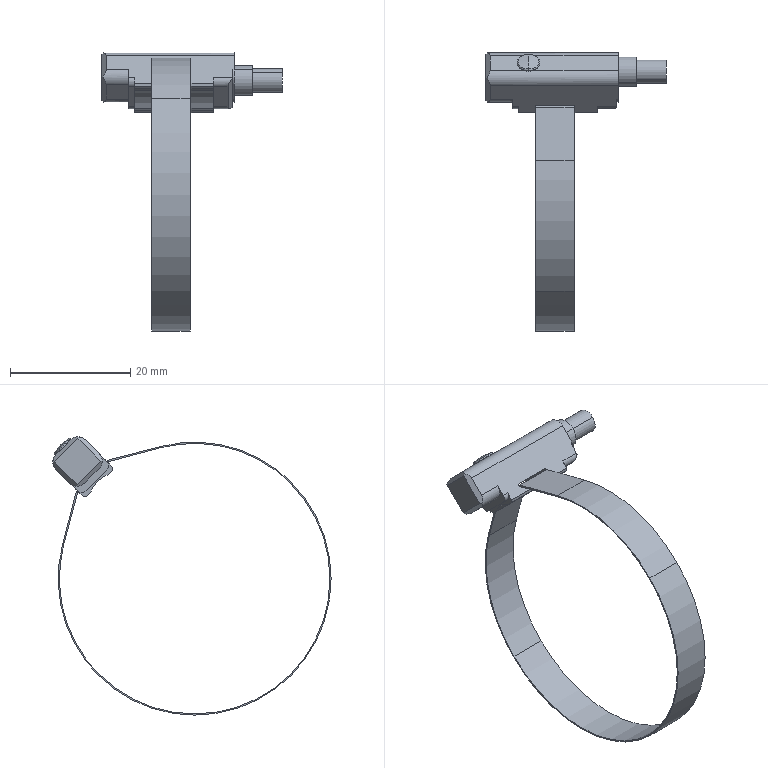Component | SolidWorks | CS1_M_A40-1 | 1 solid | 66 faces | box 30 x 46.28 x 46.28 mm | volume 1437 mm3 | plane 37 | cylinder 25 | sphere 2 | torus 2 | commonest cylinder face diameters 3.4 x6 45 x5 2 x4 45.4 x3 3.8 x2 3.9 x2 4.9 x2 10 x1
build123d program:
from build123d import *

# Parameters (mm, degrees)
EXTRUDE1_DEPTH              = 3.175
EXTRUDE1_DEPTH_BACK         = 3.175
EXTRUDE2_DEPTH              = 18.5
EXTRUDE3_DEPTH              = 4.5
EXTRUDE4_DEPTH              = 5.5
EXTRUDE5_DEPTH              = 18.5
EXTRUDE6_DEPTH              = 3.5
EXTRUDE7_DEPTH              = 3.25
EXTRUDE7_DEPTH_BACK         = 3.25
SKETCH7_W                   = 7.3
SKETCH7_H                   = 0.3
SKETCH8_R                   = 2.45
EXTRUDE8_DEPTH              = 25
SKETCH9_R                   = 1.95
EXTRUDE9_DEPTH              = 30
EXTRUDE10_DEPTH             = 3.2
EXTRUDE11_DEPTH             = 5
EXTRUDE11_DEPTH_BACK        = 5
EXTRUDE12_DEPTH             = 5
EXTRUDE12_DEPTH_BACK        = 5
EXTRUDE13_DEPTH             = 10
EXTRUDE13_DEPTH_BACK        = 10
TUBESADDLERELIEF_DEPTH      = 50.067
TUBESADDLERELIEF_DEPTH_BACK = 50.067
SKETCH15_R                  = 22.5


with BuildPart() as part:
    # Sketch1 → Extrude1 (new, two sides: drawn at the far end of the back side and taken through both)
    with BuildSketch(Plane(origin=(11.5, 0, 0), x_dir=(0, 0, -1), z_dir=(1, 0, 0)).offset(-EXTRUDE1_DEPTH_BACK)):
        with BuildLine():
            Line((11.53, 19.554), (3.65, 24.2))
            Line((3.65, 24.2), (-3.65, 24.2))
            Line((-3.65, 24.2), (-11.53, 19.554))
            ThreePointArc((-11.53, 19.554), (0, -22.7), (11.53, 19.554))
        make_face()
        with BuildLine():
            Line((11.271, 19.474), (3.45, 24))
            Line((3.45, 24), (-3.45, 24))
            Line((-3.45, 24), (-11.271, 19.474))
            ThreePointArc((-11.271, 19.474), (0, -22.5), (11.271, 19.474))
        make_face(mode=Mode.SUBTRACT)
    extrude(amount=EXTRUDE1_DEPTH + EXTRUDE1_DEPTH_BACK)

    # Sketch2 → Extrude2 (add)
    with BuildSketch(Plane(origin=(0, 0, 0), x_dir=(0, 0, -1), z_dir=(1, 0, 0))):
        with BuildLine():
            Line((-3.45, 22.714), (-3.096, 22.361))
            Line((-3.096, 22.361), (-2.5, 22.361))
            Line((-2.5, 22.361), (-2.5, 21.8))
            Line((-2.5, 21.8), (2.5, 21.8))
            Line((2.5, 21.8), (2.5, 22.361))
            Line((2.5, 22.361), (3.096, 22.361))
            Line((3.096, 22.361), (3.45, 22.714))
            Line((3.45, 22.714), (3.45, 29.2))
            ThreePointArc((3.45, 29.2), (2.952, 30.402), (1.75, 30.9))
            Line((1.75, 30.9), (-1.75, 30.9))
            ThreePointArc((-1.75, 30.9), (-2.952, 30.402), (-3.45, 29.2))
            Line((-3.45, 29.2), (-3.45, 22.714))
        make_face()
    extrude(amount=EXTRUDE2_DEPTH)

    # Sketch3 → Extrude3 (cut)
    with BuildSketch(Plane(origin=(0, 0, 0), x_dir=(0, 0, -1), z_dir=(1, 0, 0))):
        with BuildLine():
            Line((-3.45, 25.9), (-3.45, 22.714))
            Line((-3.45, 22.714), (-3.096, 22.361))
            Line((-3.096, 22.361), (-2.5, 22.361))
            Line((-2.5, 22.361), (-2.5, 21.8))
            Line((-2.5, 21.8), (2.5, 21.8))
            Line((2.5, 21.8), (2.5, 22.361))
            Line((2.5, 22.361), (3.096, 22.361))
            Line((3.096, 22.361), (3.45, 22.714))
            Line((3.45, 22.714), (3.45, 25.9))
            ThreePointArc((3.45, 25.9), (2.952, 24.698), (1.75, 24.2))
            Line((1.75, 24.2), (-1.75, 24.2))
            ThreePointArc((-1.75, 24.2), (-2.952, 24.698), (-3.45, 25.9))
        make_face()
    extrude(amount=EXTRUDE3_DEPTH, mode=Mode.SUBTRACT)

    # Sketch4 → Extrude4 (cut)
    with BuildSketch(Plane(origin=(0, 0, 0), x_dir=(0, 0, -1), z_dir=(1, 0, 0))):
        with BuildLine():
            Line((-3.45, 22.714), (-3.096, 22.361))
            Line((-3.096, 22.361), (-2.5, 22.361))
            Line((-2.5, 22.361), (-2.5, 21.8))
            Line((-2.5, 21.8), (2.5, 21.8))
            Line((2.5, 21.8), (2.5, 22.361))
            Line((2.5, 22.361), (3.096, 22.361))
            Line((3.096, 22.361), (3.45, 22.714))
            Line((3.45, 22.714), (3.45, 24.1))
            ThreePointArc((3.45, 24.1), (3.157, 23.393), (2.45, 23.1))
            Line((2.45, 23.1), (-2.45, 23.1))
            ThreePointArc((-2.45, 23.1), (-3.157, 23.393), (-3.45, 24.1))
            Line((-3.45, 24.1), (-3.45, 22.714))
        make_face()
    extrude(amount=EXTRUDE4_DEPTH, mode=Mode.SUBTRACT)

    # Sketch5 → Extrude5 (cut)
    with BuildSketch(Plane(origin=(0, 0, 0), x_dir=(0, 0, -1), z_dir=(1, 0, 0))):
        with BuildLine():
            Line((-2.5, 21.4), (2.5, 21.4))
            Line((2.5, 21.4), (2.5, 22.361))
            Line((2.5, 22.361), (2.18, 22.361))
            ThreePointArc((2.18, 22.361), (0, 22.861), (-2.18, 22.361))
            Line((-2.18, 22.361), (-2.5, 22.361))
            Line((-2.5, 22.361), (-2.5, 21.4))
        make_face()
    extrude(amount=EXTRUDE5_DEPTH, mode=Mode.SUBTRACT)

    # Sketch6 → Extrude6 (add)
    with BuildSketch(Plane(origin=(18.5, 0, 0), x_dir=(0, 0, -1), z_dir=(1, 0, 0))):
        with BuildLine():
            Line((-1.75, 24.2), (1.75, 24.2))
            ThreePointArc((1.75, 24.2), (2.952, 24.698), (3.45, 25.9))
            Line((3.45, 25.9), (3.45, 29.2))
            ThreePointArc((3.45, 29.2), (2.952, 30.402), (1.75, 30.9))
            Line((1.75, 30.9), (-1.75, 30.9))
            ThreePointArc((-1.75, 30.9), (-2.952, 30.402), (-3.45, 29.2))
            Line((-3.45, 29.2), (-3.45, 25.9))
            ThreePointArc((-3.45, 25.9), (-2.952, 24.698), (-1.75, 24.2))
        make_face()
    extrude(amount=EXTRUDE6_DEPTH)

    # Sketch7 → Extrude7 (cut, two sides: drawn at the far end of the back side and taken through both)
    with BuildSketch(Plane(origin=(11.5, 0, 0), x_dir=(0, 0, -1), z_dir=(1, 0, 0)).offset(-EXTRUDE7_DEPTH_BACK)):
        with Locations((0, 24.35)):
            Rectangle(SKETCH7_W, SKETCH7_H)
    extrude(amount=EXTRUDE7_DEPTH + EXTRUDE7_DEPTH_BACK, mode=Mode.SUBTRACT)

    # Sketch8 → Extrude8 (add)
    with BuildSketch(Plane(origin=(0, 0, 0), x_dir=(0, 0, -1), z_dir=(1, 0, 0))):
        with Locations((1, 27.9)):
            Circle(SKETCH8_R)
    extrude(amount=EXTRUDE8_DEPTH)

    # Sketch9 → Extrude9 (add)
    with BuildSketch(Plane(origin=(0, 0, 0), x_dir=(0, 0, -1), z_dir=(1, 0, 0))):
        with Locations((1, 27.9)):
            Circle(SKETCH9_R)
    extrude(amount=EXTRUDE9_DEPTH)

    # Sketch10 → Extrude10 (add)
    with BuildSketch(Plane(origin=(18.5, 0, 0), x_dir=(0, 0, -1), z_dir=(1, 0, 0))):
        with BuildLine():
            Line((-3.45, 25.9), (-3.45, 24.1))
            ThreePointArc((-3.45, 24.1), (-3.157, 23.393), (-2.45, 23.1))
            Line((-2.45, 23.1), (2.45, 23.1))
            ThreePointArc((2.45, 23.1), (3.157, 23.393), (3.45, 24.1))
            Line((3.45, 24.1), (3.45, 25.9))
            ThreePointArc((3.45, 25.9), (2.952, 24.698), (1.75, 24.2))
            Line((1.75, 24.2), (-1.75, 24.2))
            ThreePointArc((-1.75, 24.2), (-2.952, 24.698), (-3.45, 25.9))
        make_face()
    extrude(amount=EXTRUDE10_DEPTH)

    # Sketch11 → Extrude11 (cut, two sides: drawn at the far end of the back side and taken through both)
    with BuildSketch(Plane.XY.offset(-EXTRUDE11_DEPTH_BACK)):
        Polygon((20.993, 23.1), (20.993, 22.1), (22.7, 22.1), (22.7, 23.807), (21.7, 23.807), align=None)
    extrude(amount=EXTRUDE11_DEPTH + EXTRUDE11_DEPTH_BACK, mode=Mode.SUBTRACT)

    # Sketch12 → Extrude12 (cut, two sides: drawn at the far end of the back side and taken through both)
    with BuildSketch(Plane.XY.offset(-EXTRUDE12_DEPTH_BACK)):
        Polygon((-1, 31.9), (-1, 23.2), (0.7071, 23.2), (0.7071, 24.2), (0, 24.907), (0, 30.193), (0.7071, 30.9), (0.7071, 31.9), align=None)
    extrude(amount=EXTRUDE12_DEPTH + EXTRUDE12_DEPTH_BACK, mode=Mode.SUBTRACT)

    # Sketch13 → Extrude13 (cut, two sides: drawn at the far end of the back side and taken through both)
    with BuildSketch(Plane(origin=(0, 30.9, 0), x_dir=(1, 0, 0), z_dir=(0, 1, 0)).offset(-EXTRUDE13_DEPTH_BACK)):
        Polygon((-1, -4.45), (0.7071, -4.45), (0.7071, -3.45), (0, -2.743), (0, 2.743), (0.7071, 3.45), (0.7071, 4.45), (-1, 4.45), align=None)
    extrude(amount=EXTRUDE13_DEPTH + EXTRUDE13_DEPTH_BACK, mode=Mode.SUBTRACT)

    # Sketch14 → Revolve1 (revolve)
    with BuildSketch(Plane(origin=(7.1, 0, 0), x_dir=(0, 0, -1), z_dir=(1, 0, 0)), mode=Mode.PRIVATE) as revolve1_sk:
        with BuildLine():
            Line((0, 30.9), (-1.9, 30.9))
            Line((-1.9, 30.9), (-1.9, 31.015))
            ThreePointArc((-1.9, 31.015), (-1.85, 31.166), (-1.72, 31.256))
            ThreePointArc((-1.72, 31.256), (-0.8685, 31.439), (0, 31.5))
            Line((0, 31.5), (0, 30.9))
        make_face()
    revolve(revolve1_sk.sketch.rotate(Axis((7.1, 31.5, 0), (0, -1, 0)), 180), axis=Axis((7.1, 31.5, 0), (0, -1, 0)))

    # Sketch15 → TubeSaddleRelief (cut, two sides: drawn at the far end of the back side and taken through both)
    with BuildSketch(Plane(origin=(0, 0, 0), x_dir=(0, 0, -1), z_dir=(1, 0, 0)).offset(-TUBESADDLERELIEF_DEPTH_BACK)):
        Circle(SKETCH15_R)
    extrude(amount=TUBESADDLERELIEF_DEPTH + TUBESADDLERELIEF_DEPTH_BACK, mode=Mode.SUBTRACT)


solid = part.part

# Placed as in the assembly
solid = solid.moved(Location((23, 0, 0), (45, 0, 0)))